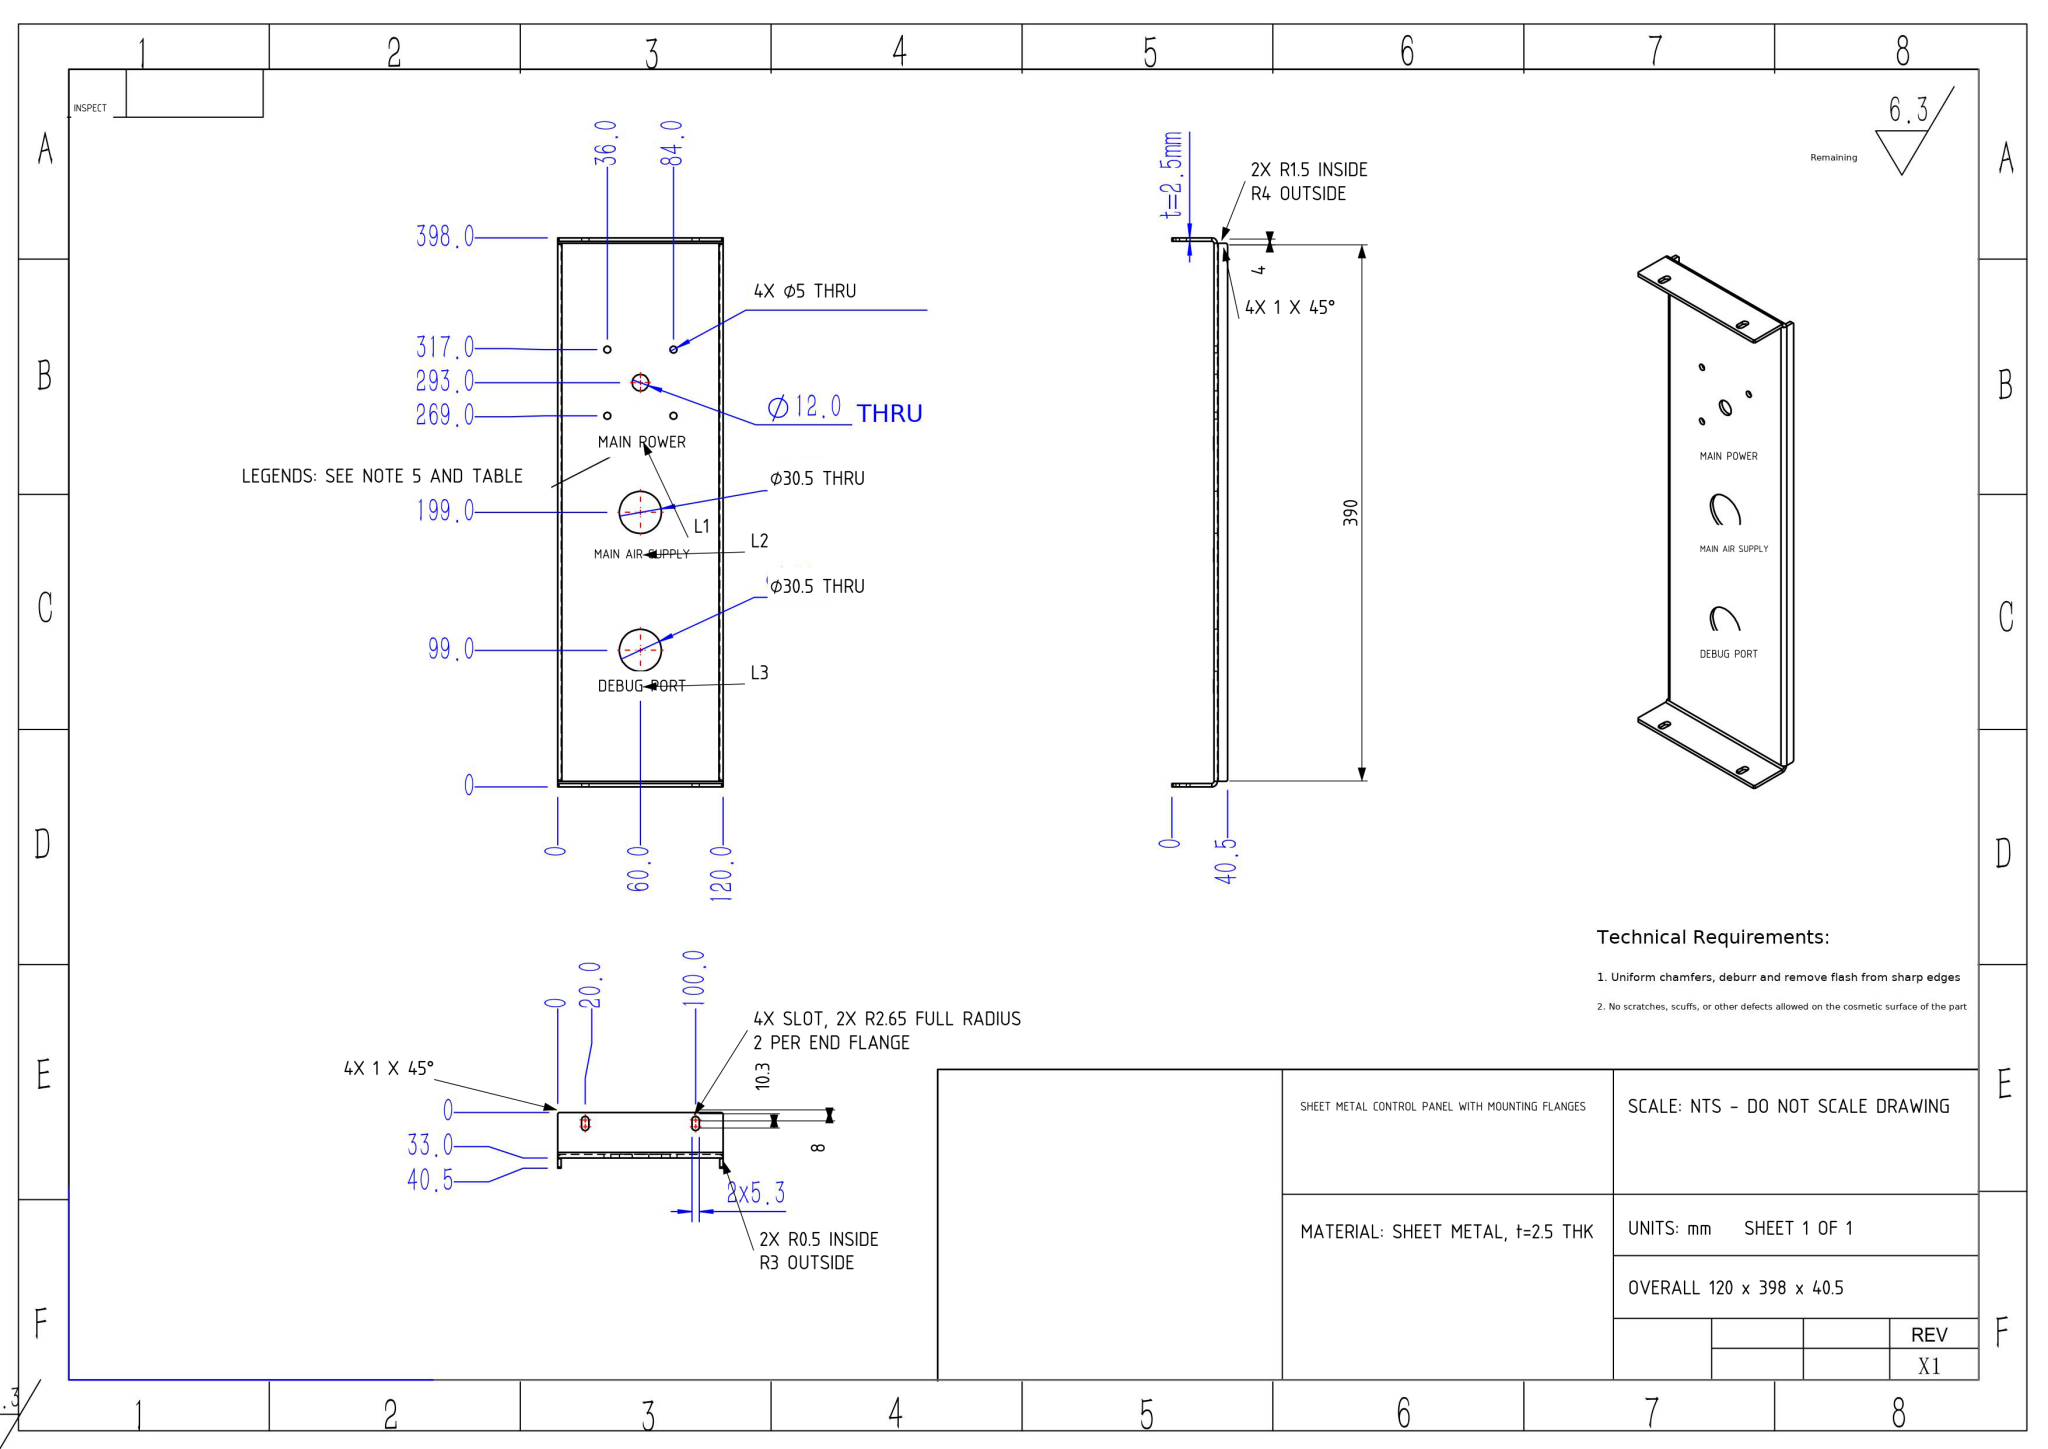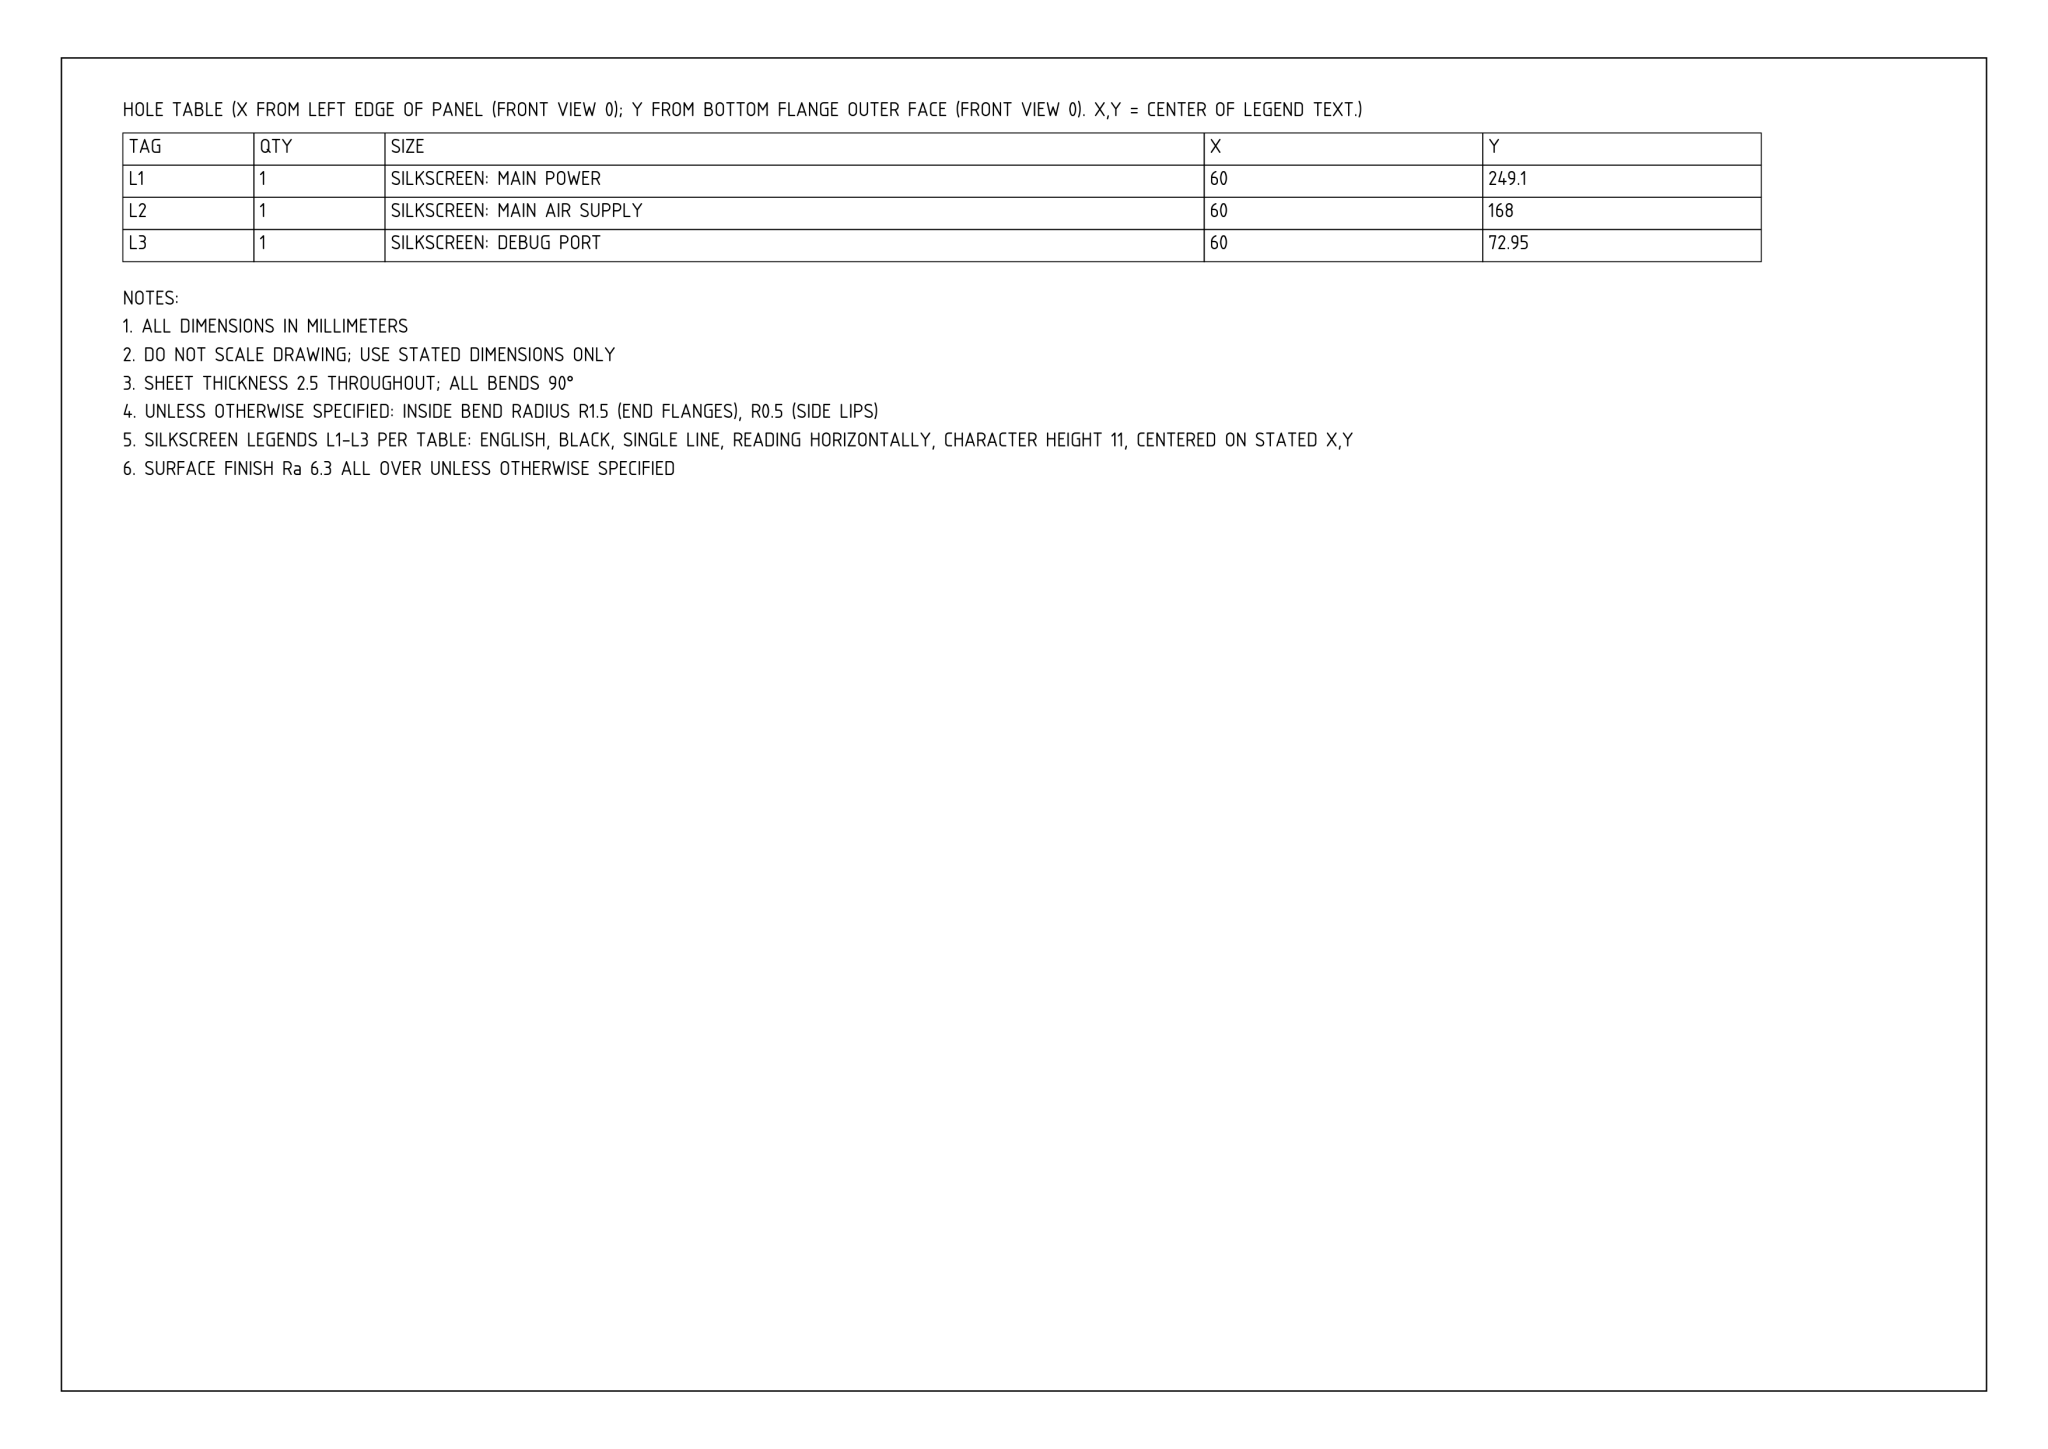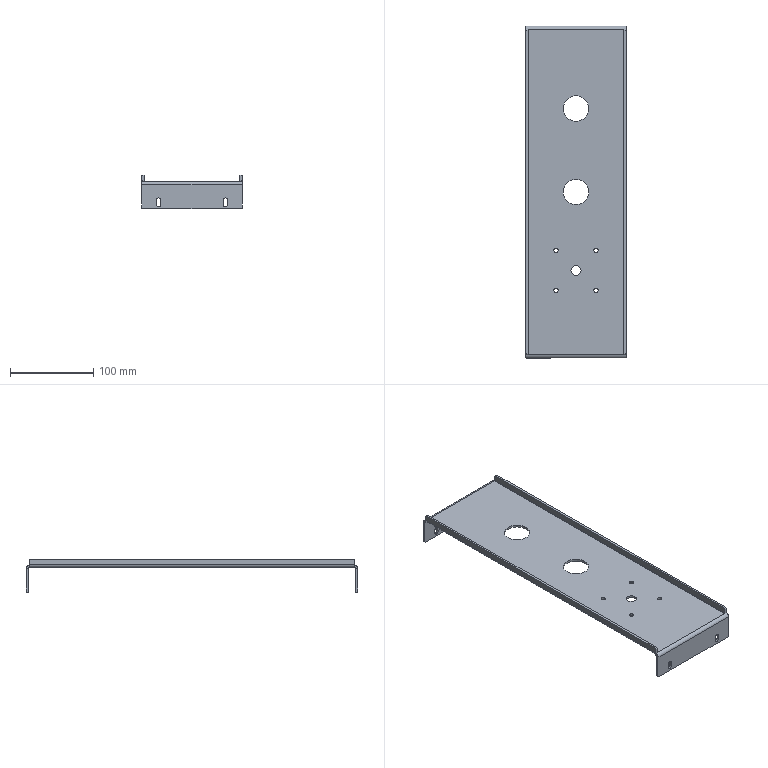Part | NX | mm | 1 solid | 587 faces | box 120 x 398 x 40.5 mm | volume 145543 mm3 | plane 393 | spline 160 | cylinder 34 | commonest cylinder face diameters 5.3 x12 5 x8 30.5 x4 12 x2 8 x2 3 x2 6 x2 1 x2